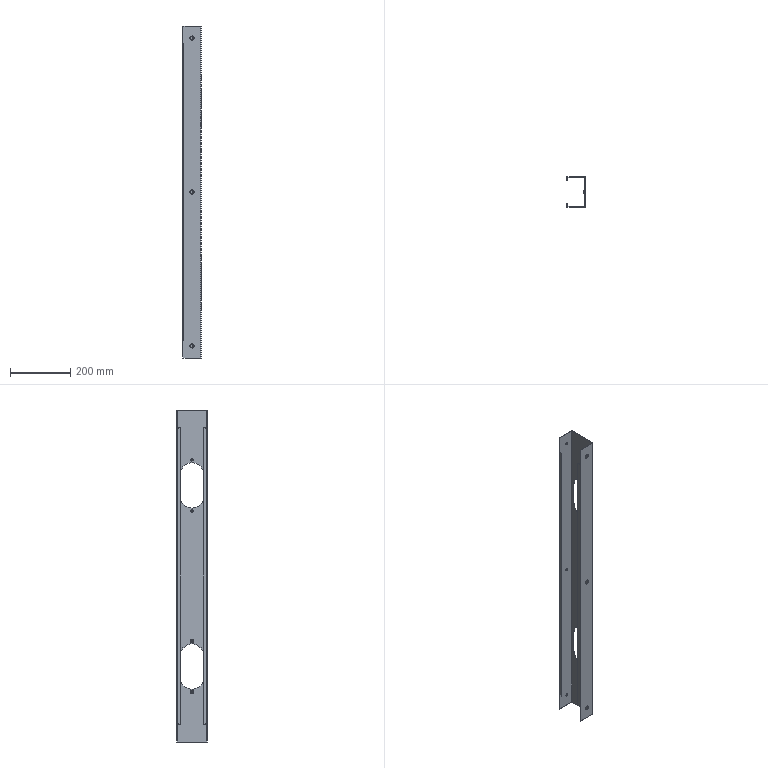Component | SolidWorks | BaseWeldment-1_BottomFrameRear-1 | 1 solid | 94 faces | volume 354214 mm3 | cylinder 52 | plane 38 | spline 4 | commonest cylinder face diameters 4 x10 8 x8 14 x6 8.5 x6 80 x6 6 x4 11 x4 0.2 x4